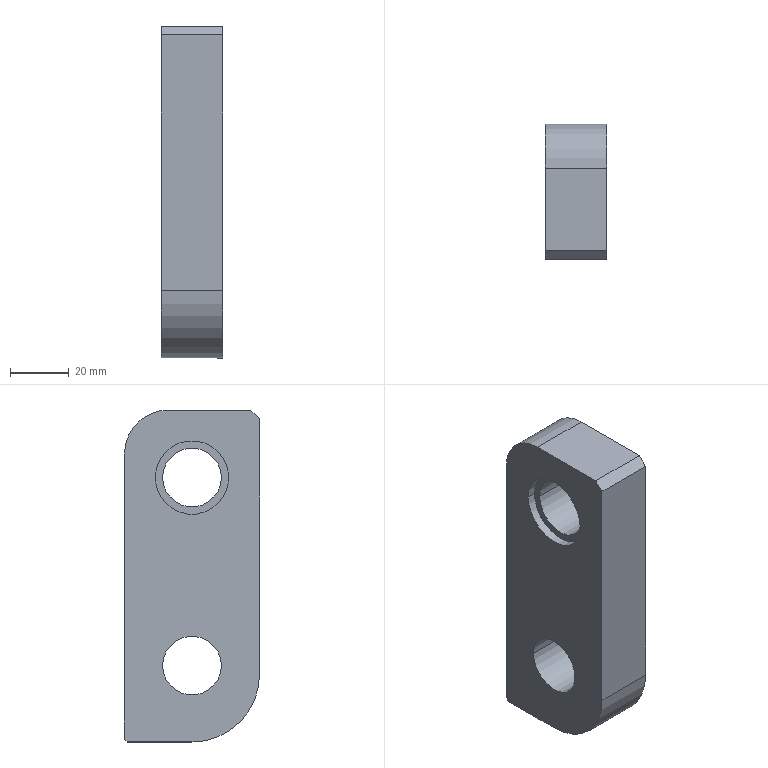Component | SolidWorks | GL9-255--p_O(_k)-1 | 1 solid | 17 faces | box 21 x 46 x 113 mm | volume 91930 mm3 | plane 9 | cylinder 8 | commonest cylinder face diameters 20 x4 25 x2 30 x1 46 x1
build123d program:
from build123d import *

# Parameters (mm, degrees)
SKETCH1_W      = 113
SKETCH1_H      = 46
EXTRUDE1_DEPTH = 21
FILLET1_R      = 15
FILLET2_R      = 23
SKETCH2_R      = 10
EXTRUDE2_DEPTH = 124.798
CHAMFER1_SIZE  = 3
CHAMFER2_SIZE  = 1
SKETCH4_R      = 12.5
EXTRUDE4_DEPTH = 3
SKETCH5_R      = 10
EXTRUDE5_DEPTH = 124.325


with BuildPart() as part:
    # Sketch1 → Extrude1 (new body)
    with BuildSketch(Plane(origin=(0, 0, 0), x_dir=(1, 0, 0), z_dir=(0, 1, 0))):
        with Locations((-56.5, -23)):
            Rectangle(SKETCH1_W, SKETCH1_H)
    extrude(amount=EXTRUDE1_DEPTH)

    # Fillet1
    fillet1_edges = [part.edges().sort_by_distance(p)[0] for p in [
        (-113, 10.5, 0),
    ]]
    fillet(fillet1_edges, radius=FILLET1_R)

    # Fillet2
    fillet2_edges = [part.edges().sort_by_distance(p)[0] for p in [
        (0, 10.5, 46),
    ]]
    fillet(fillet2_edges, radius=FILLET2_R)

    # Sketch2 → Extrude2 (cut, through all)
    with BuildSketch(Plane(origin=(0, 21, 0), x_dir=(1, 0, 0), z_dir=(0, 1, 0))):
        with Locations(Location((-26, -23, 0), (0, 0, 270))):
            Circle(SKETCH2_R)
    extrude(amount=-EXTRUDE2_DEPTH, mode=Mode.SUBTRACT)

    # Chamfer1
    chamfer1_edges = [part.edges().sort_by_distance(p)[0] for p in [
        (-113, 10.5, 46),
    ]]
    chamfer(chamfer1_edges, length=CHAMFER1_SIZE)

    # Chamfer2
    chamfer2_edges = [part.edges().sort_by_distance(p)[0] for p in [
        (0, 10.5, 0),
    ]]
    chamfer(chamfer2_edges, length=CHAMFER2_SIZE)

    # Sketch4 → Extrude4 (cut)
    with BuildSketch(Plane.XZ):
        with Locations(Location((-90, 23, 0), (0, 0, 270))):
            Circle(SKETCH4_R)
    extrude(amount=-EXTRUDE4_DEPTH, mode=Mode.SUBTRACT)

    # Sketch5 → Extrude5 (cut, through all)
    with BuildSketch(Plane.XZ.offset(-3)):
        with Locations(Location((-90, 23, 0), (0, 0, 270))):
            Circle(SKETCH5_R)
    extrude(amount=-EXTRUDE5_DEPTH, mode=Mode.SUBTRACT)


solid = part.part

# Placed as in the assembly
solid = solid.moved(Location((64, 104, -550), (90, 0, -90)))
STEP:
#1=COLOUR_RGB('',0.7922,0.8196,0.9333);
#2=FILL_AREA_STYLE_COLOUR('',#1);
#3=FILL_AREA_STYLE('',(#2));
#4=SURFACE_STYLE_FILL_AREA(#3);
#5=SURFACE_SIDE_STYLE('',(#4));
#6=SURFACE_STYLE_USAGE(.BOTH.,#5);
#7=PRESENTATION_STYLE_ASSIGNMENT((#6));
#8=CARTESIAN_POINT('',(3.346,2.795,-18.11));
#9=VERTEX_POINT('',#8);
#10=CARTESIAN_POINT('',(3.346,3.583,-18.11));
#11=VERTEX_POINT('',#10);
#12=CARTESIAN_POINT('',(3.346,3.189,-18.11));
#13=DIRECTION('',(-1.,0.,0.));
#14=DIRECTION('',(0.,1.,0.));
#15=AXIS2_PLACEMENT_3D('',#12,#13,#14);
#16=CIRCLE('',#15,0.3937);
#17=EDGE_CURVE('',#9,#11,#16,.T.);
#18=ORIENTED_EDGE('',*,*,#17,.F.);
#19=CARTESIAN_POINT('',(2.638,2.795,-18.11));
#20=VERTEX_POINT('',#19);
#21=CARTESIAN_POINT('',(3.346,2.795,-18.11));
#22=DIRECTION('',(-1.,0.,0.));
#23=VECTOR('',#22,39.37);
#24=LINE('',#21,#23);
#25=EDGE_CURVE('',#9,#20,#24,.T.);
#26=ORIENTED_EDGE('',*,*,#25,.T.);
#27=CARTESIAN_POINT('',(2.638,3.583,-18.11));
#28=VERTEX_POINT('',#27);
#29=CARTESIAN_POINT('',(2.638,3.189,-18.11));
#30=DIRECTION('',(-1.,0.,0.));
#31=DIRECTION('',(0.,1.,0.));
#32=AXIS2_PLACEMENT_3D('',#29,#30,#31);
#33=CIRCLE('',#32,0.3937);
#34=EDGE_CURVE('',#20,#28,#33,.T.);
#35=ORIENTED_EDGE('',*,*,#34,.T.);
#36=CARTESIAN_POINT('',(3.346,3.583,-18.11));
#37=DIRECTION('',(-1.,0.,0.));
#38=VECTOR('',#37,39.37);
#39=LINE('',#36,#38);
#40=EDGE_CURVE('',#11,#28,#39,.T.);
#41=ORIENTED_EDGE('',*,*,#40,.F.);
#42=EDGE_LOOP('',(#18,#26,#35,#41));
#43=FACE_OUTER_BOUND('',#42,.T.);
#44=CARTESIAN_POINT('',(3.346,3.189,-18.11));
#45=DIRECTION('',(-1.,0.,0.));
#46=DIRECTION('',(0.,1.,0.));
#47=AXIS2_PLACEMENT_3D('',#44,#45,#46);
#48=CYLINDRICAL_SURFACE('',#47,0.3937);
#49=ADVANCED_FACE('',(#43),#48,.F.);
#50=CARTESIAN_POINT('',(2.638,2.697,-18.11));
#51=VERTEX_POINT('',#50);
#52=CARTESIAN_POINT('',(2.638,3.681,-18.11));
#53=VERTEX_POINT('',#52);
#54=CARTESIAN_POINT('',(2.638,3.189,-18.11));
#55=DIRECTION('',(-1.,0.,0.));
#56=DIRECTION('',(0.,1.,0.));
#57=AXIS2_PLACEMENT_3D('',#54,#55,#56);
#58=CIRCLE('',#57,0.4921);
#59=EDGE_CURVE('',#51,#53,#58,.T.);
#60=ORIENTED_EDGE('',*,*,#59,.F.);
#61=CARTESIAN_POINT('',(2.52,2.697,-18.11));
#62=VERTEX_POINT('',#61);
#63=CARTESIAN_POINT('',(2.638,2.697,-18.11));
#64=DIRECTION('',(-1.,0.,0.));
#65=VECTOR('',#64,39.37);
#66=LINE('',#63,#65);
#67=EDGE_CURVE('',#51,#62,#66,.T.);
#68=ORIENTED_EDGE('',*,*,#67,.T.);
#69=CARTESIAN_POINT('',(2.52,3.681,-18.11));
#70=VERTEX_POINT('',#69);
#71=CARTESIAN_POINT('',(2.52,3.189,-18.11));
#72=DIRECTION('',(-1.,0.,0.));
#73=DIRECTION('',(0.,1.,0.));
#74=AXIS2_PLACEMENT_3D('',#71,#72,#73);
#75=CIRCLE('',#74,0.4921);
#76=EDGE_CURVE('',#62,#70,#75,.T.);
#77=ORIENTED_EDGE('',*,*,#76,.T.);
#78=CARTESIAN_POINT('',(2.638,3.681,-18.11));
#79=DIRECTION('',(-1.,0.,0.));
#80=VECTOR('',#79,39.37);
#81=LINE('',#78,#80);
#82=EDGE_CURVE('',#53,#70,#81,.T.);
#83=ORIENTED_EDGE('',*,*,#82,.F.);
#84=EDGE_LOOP('',(#60,#68,#77,#83));
#85=FACE_OUTER_BOUND('',#84,.T.);
#86=CARTESIAN_POINT('',(2.638,3.189,-18.11));
#87=DIRECTION('',(-1.,0.,0.));
#88=DIRECTION('',(0.,1.,0.));
#89=AXIS2_PLACEMENT_3D('',#86,#87,#88);
#90=CYLINDRICAL_SURFACE('',#89,0.4921);
#91=ADVANCED_FACE('',(#85),#90,.F.);
#92=CARTESIAN_POINT('',(2.52,3.583,-20.63));
#93=VERTEX_POINT('',#92);
#94=CARTESIAN_POINT('',(2.52,2.795,-20.63));
#95=VERTEX_POINT('',#94);
#96=CARTESIAN_POINT('',(2.52,3.189,-20.63));
#97=DIRECTION('',(1.,-0.,-0.));
#98=DIRECTION('',(0.,-1.,0.));
#99=AXIS2_PLACEMENT_3D('',#96,#97,#98);
#100=CIRCLE('',#99,0.3937);
#101=EDGE_CURVE('',#93,#95,#100,.T.);
#102=ORIENTED_EDGE('',*,*,#101,.F.);
#103=CARTESIAN_POINT('',(3.346,3.583,-20.63));
#104=VERTEX_POINT('',#103);
#105=CARTESIAN_POINT('',(2.52,3.583,-20.63));
#106=DIRECTION('',(1.,-0.,-0.));
#107=VECTOR('',#106,39.37);
#108=LINE('',#105,#107);
#109=EDGE_CURVE('',#93,#104,#108,.T.);
#110=ORIENTED_EDGE('',*,*,#109,.T.);
#111=CARTESIAN_POINT('',(3.346,2.795,-20.63));
#112=VERTEX_POINT('',#111);
#113=CARTESIAN_POINT('',(3.346,3.189,-20.63));
#114=DIRECTION('',(1.,-0.,-0.));
#115=DIRECTION('',(0.,-1.,0.));
#116=AXIS2_PLACEMENT_3D('',#113,#114,#115);
#117=CIRCLE('',#116,0.3937);
#118=EDGE_CURVE('',#104,#112,#117,.T.);
#119=ORIENTED_EDGE('',*,*,#118,.T.);
#120=CARTESIAN_POINT('',(2.52,2.795,-20.63));
#121=DIRECTION('',(1.,-0.,-0.));
#122=VECTOR('',#121,39.37);
#123=LINE('',#120,#122);
#124=EDGE_CURVE('',#95,#112,#123,.T.);
#125=ORIENTED_EDGE('',*,*,#124,.F.);
#126=EDGE_LOOP('',(#102,#110,#119,#125));
#127=FACE_OUTER_BOUND('',#126,.T.);
#128=CARTESIAN_POINT('',(2.52,3.189,-20.63));
#129=DIRECTION('',(1.,-0.,-0.));
#130=DIRECTION('',(0.,-1.,0.));
#131=AXIS2_PLACEMENT_3D('',#128,#129,#130);
#132=CYLINDRICAL_SURFACE('',#131,0.3937);
#133=ADVANCED_FACE('',(#127),#132,.F.);
#134=CARTESIAN_POINT('',(2.52,3.189,-21.654));
#135=VERTEX_POINT('',#134);
#136=CARTESIAN_POINT('',(2.52,4.055,-21.654));
#137=VERTEX_POINT('',#136);
#138=CARTESIAN_POINT('',(2.52,2.283,-21.654));
#139=DIRECTION('',(0.,1.,0.));
#140=VECTOR('',#139,39.37);
#141=LINE('',#138,#140);
#142=EDGE_CURVE('',#135,#137,#141,.T.);
#143=ORIENTED_EDGE('',*,*,#142,.T.);
#144=CARTESIAN_POINT('',(3.346,4.055,-21.654));
#145=VERTEX_POINT('',#144);
#146=CARTESIAN_POINT('',(3.346,4.055,-21.654));
#147=DIRECTION('',(1.,-0.,-0.));
#148=VECTOR('',#147,39.37);
#149=LINE('',#146,#148);
#150=EDGE_CURVE('',#137,#145,#149,.T.);
#151=ORIENTED_EDGE('',*,*,#150,.T.);
#152=CARTESIAN_POINT('',(3.346,3.189,-21.654));
#153=VERTEX_POINT('',#152);
#154=CARTESIAN_POINT('',(3.346,2.283,-21.654));
#155=DIRECTION('',(0.,1.,0.));
#156=VECTOR('',#155,39.37);
#157=LINE('',#154,#156);
#158=EDGE_CURVE('',#153,#145,#157,.T.);
#159=ORIENTED_EDGE('',*,*,#158,.F.);
#160=CARTESIAN_POINT('',(3.346,3.189,-21.654));
#161=DIRECTION('',(-1.,0.,0.));
#162=VECTOR('',#161,39.37);
#163=LINE('',#160,#162);
#164=EDGE_CURVE('',#153,#135,#163,.T.);
#165=ORIENTED_EDGE('',*,*,#164,.T.);
#166=EDGE_LOOP('',(#143,#151,#159,#165));
#167=FACE_OUTER_BOUND('',#166,.T.);
#168=CARTESIAN_POINT('',(3.346,2.283,-21.654));
#169=DIRECTION('',(0.,-0.,1.));
#170=DIRECTION('',(-0.,-1.,-0.));
#171=AXIS2_PLACEMENT_3D('',#168,#169,#170);
#172=PLANE('',#171);
#173=ADVANCED_FACE('',(#167),#172,.F.);
#174=CARTESIAN_POINT('',(3.346,4.094,-21.614));
#175=VERTEX_POINT('',#174);
#176=CARTESIAN_POINT('',(3.346,4.094,-17.795));
#177=VERTEX_POINT('',#176);
#178=CARTESIAN_POINT('',(3.346,4.094,-21.654));
#179=DIRECTION('',(0.,-0.,1.));
#180=VECTOR('',#179,39.37);
#181=LINE('',#178,#180);
#182=EDGE_CURVE('',#175,#177,#181,.T.);
#183=ORIENTED_EDGE('',*,*,#182,.F.);
#184=CARTESIAN_POINT('',(2.52,4.094,-21.614));
#185=VERTEX_POINT('',#184);
#186=CARTESIAN_POINT('',(3.346,4.094,-21.614));
#187=DIRECTION('',(-1.,0.,0.));
#188=VECTOR('',#187,39.37);
#189=LINE('',#186,#188);
#190=EDGE_CURVE('',#175,#185,#189,.T.);
#191=ORIENTED_EDGE('',*,*,#190,.T.);
#192=CARTESIAN_POINT('',(2.52,4.094,-17.795));
#193=VERTEX_POINT('',#192);
#194=CARTESIAN_POINT('',(2.52,4.094,-21.654));
#195=DIRECTION('',(0.,-0.,1.));
#196=VECTOR('',#195,39.37);
#197=LINE('',#194,#196);
#198=EDGE_CURVE('',#185,#193,#197,.T.);
#199=ORIENTED_EDGE('',*,*,#198,.T.);
#200=CARTESIAN_POINT('',(3.346,4.094,-17.795));
#201=DIRECTION('',(1.,-0.,-0.));
#202=VECTOR('',#201,39.37);
#203=LINE('',#200,#202);
#204=EDGE_CURVE('',#193,#177,#203,.T.);
#205=ORIENTED_EDGE('',*,*,#204,.T.);
#206=EDGE_LOOP('',(#183,#191,#199,#205));
#207=FACE_OUTER_BOUND('',#206,.T.);
#208=CARTESIAN_POINT('',(3.346,4.094,-21.654));
#209=DIRECTION('',(-0.,-1.,-0.));
#210=DIRECTION('',(-0.,0.,-1.));
#211=AXIS2_PLACEMENT_3D('',#208,#209,#210);
#212=PLANE('',#211);
#213=ADVANCED_FACE('',(#207),#212,.F.);
#214=CARTESIAN_POINT('',(2.52,3.504,-17.205));
#215=VERTEX_POINT('',#214);
#216=CARTESIAN_POINT('',(2.52,2.402,-17.205));
#217=VERTEX_POINT('',#216);
#218=CARTESIAN_POINT('',(2.52,4.094,-17.205));
#219=DIRECTION('',(-0.,-1.,-0.));
#220=VECTOR('',#219,39.37);
#221=LINE('',#218,#220);
#222=EDGE_CURVE('',#215,#217,#221,.T.);
#223=ORIENTED_EDGE('',*,*,#222,.T.);
#224=CARTESIAN_POINT('',(3.346,2.402,-17.205));
#225=VERTEX_POINT('',#224);
#226=CARTESIAN_POINT('',(3.346,2.402,-17.205));
#227=DIRECTION('',(1.,-0.,-0.));
#228=VECTOR('',#227,39.37);
#229=LINE('',#226,#228);
#230=EDGE_CURVE('',#217,#225,#229,.T.);
#231=ORIENTED_EDGE('',*,*,#230,.T.);
#232=CARTESIAN_POINT('',(3.346,3.504,-17.205));
#233=VERTEX_POINT('',#232);
#234=CARTESIAN_POINT('',(3.346,4.094,-17.205));
#235=DIRECTION('',(-0.,-1.,-0.));
#236=VECTOR('',#235,39.37);
#237=LINE('',#234,#236);
#238=EDGE_CURVE('',#233,#225,#237,.T.);
#239=ORIENTED_EDGE('',*,*,#238,.F.);
#240=CARTESIAN_POINT('',(3.346,3.504,-17.205));
#241=DIRECTION('',(-1.,0.,0.));
#242=VECTOR('',#241,39.37);
#243=LINE('',#240,#242);
#244=EDGE_CURVE('',#233,#215,#243,.T.);
#245=ORIENTED_EDGE('',*,*,#244,.T.);
#246=EDGE_LOOP('',(#223,#231,#239,#245));
#247=FACE_OUTER_BOUND('',#246,.T.);
#248=CARTESIAN_POINT('',(3.346,4.094,-17.205));
#249=DIRECTION('',(-0.,0.,-1.));
#250=DIRECTION('',(0.,1.,0.));
#251=AXIS2_PLACEMENT_3D('',#248,#249,#250);
#252=PLANE('',#251);
#253=ADVANCED_FACE('',(#247),#252,.F.);
#254=CARTESIAN_POINT('',(3.346,2.283,-17.323));
#255=VERTEX_POINT('',#254);
#256=CARTESIAN_POINT('',(3.346,2.283,-20.748));
#257=VERTEX_POINT('',#256);
#258=CARTESIAN_POINT('',(3.346,2.283,-17.205));
#259=DIRECTION('',(-0.,0.,-1.));
#260=VECTOR('',#259,39.37);
#261=LINE('',#258,#260);
#262=EDGE_CURVE('',#255,#257,#261,.T.);
#263=ORIENTED_EDGE('',*,*,#262,.F.);
#264=CARTESIAN_POINT('',(2.52,2.283,-17.323));
#265=VERTEX_POINT('',#264);
#266=CARTESIAN_POINT('',(3.346,2.283,-17.323));
#267=DIRECTION('',(-1.,0.,0.));
#268=VECTOR('',#267,39.37);
#269=LINE('',#266,#268);
#270=EDGE_CURVE('',#255,#265,#269,.T.);
#271=ORIENTED_EDGE('',*,*,#270,.T.);
#272=CARTESIAN_POINT('',(2.52,2.283,-20.748));
#273=VERTEX_POINT('',#272);
#274=CARTESIAN_POINT('',(2.52,2.283,-17.205));
#275=DIRECTION('',(-0.,0.,-1.));
#276=VECTOR('',#275,39.37);
#277=LINE('',#274,#276);
#278=EDGE_CURVE('',#265,#273,#277,.T.);
#279=ORIENTED_EDGE('',*,*,#278,.T.);
#280=CARTESIAN_POINT('',(3.346,2.283,-20.748));
#281=DIRECTION('',(1.,-0.,-0.));
#282=VECTOR('',#281,39.37);
#283=LINE('',#280,#282);
#284=EDGE_CURVE('',#273,#257,#283,.T.);
#285=ORIENTED_EDGE('',*,*,#284,.T.);
#286=EDGE_LOOP('',(#263,#271,#279,#285));
#287=FACE_OUTER_BOUND('',#286,.T.);
#288=CARTESIAN_POINT('',(3.346,2.283,-17.205));
#289=DIRECTION('',(0.,1.,0.));
#290=DIRECTION('',(0.,-0.,1.));
#291=AXIS2_PLACEMENT_3D('',#288,#289,#290);
#292=PLANE('',#291);
#293=ADVANCED_FACE('',(#287),#292,.F.);
#294=CARTESIAN_POINT('',(3.346,3.189,-18.11));
#295=DIRECTION('',(-1.,0.,0.));
#296=DIRECTION('',(0.,1.,0.));
#297=AXIS2_PLACEMENT_3D('',#294,#295,#296);
#298=CIRCLE('',#297,0.3937);
#299=EDGE_CURVE('',#11,#9,#298,.T.);
#300=ORIENTED_EDGE('',*,*,#299,.T.);
#301=ORIENTED_EDGE('',*,*,#17,.T.);
#302=EDGE_LOOP('',(#300,#301));
#303=FACE_BOUND('',#302,.T.);
#304=CARTESIAN_POINT('',(3.346,3.189,-20.63));
#305=DIRECTION('',(1.,-0.,-0.));
#306=DIRECTION('',(0.,-1.,0.));
#307=AXIS2_PLACEMENT_3D('',#304,#305,#306);
#308=CIRCLE('',#307,0.3937);
#309=EDGE_CURVE('',#112,#104,#308,.T.);
#310=ORIENTED_EDGE('',*,*,#309,.F.);
#311=ORIENTED_EDGE('',*,*,#118,.F.);
#312=EDGE_LOOP('',(#310,#311));
#313=FACE_BOUND('',#312,.T.);
#314=ORIENTED_EDGE('',*,*,#158,.T.);
#315=CARTESIAN_POINT('',(3.346,4.075,-21.634));
#316=DIRECTION('',(0.,0.7071,0.7071));
#317=VECTOR('',#316,39.37);
#318=LINE('',#315,#317);
#319=EDGE_CURVE('',#145,#175,#318,.T.);
#320=ORIENTED_EDGE('',*,*,#319,.T.);
#321=ORIENTED_EDGE('',*,*,#182,.T.);
#322=CARTESIAN_POINT('',(3.346,3.504,-17.795));
#323=DIRECTION('',(1.,-0.,-0.));
#324=DIRECTION('',(0.,-1.,0.));
#325=AXIS2_PLACEMENT_3D('',#322,#323,#324);
#326=CIRCLE('',#325,0.5906);
#327=EDGE_CURVE('',#177,#233,#326,.T.);
#328=ORIENTED_EDGE('',*,*,#327,.T.);
#329=ORIENTED_EDGE('',*,*,#238,.T.);
#330=CARTESIAN_POINT('',(3.346,1.024,-18.583));
#331=DIRECTION('',(-0.,-0.7071,-0.7071));
#332=VECTOR('',#331,39.37);
#333=LINE('',#330,#332);
#334=EDGE_CURVE('',#225,#255,#333,.T.);
#335=ORIENTED_EDGE('',*,*,#334,.T.);
#336=ORIENTED_EDGE('',*,*,#262,.T.);
#337=CARTESIAN_POINT('',(3.346,3.189,-20.748));
#338=DIRECTION('',(1.,-0.,-0.));
#339=DIRECTION('',(0.,-1.,0.));
#340=AXIS2_PLACEMENT_3D('',#337,#338,#339);
#341=CIRCLE('',#340,0.9055);
#342=EDGE_CURVE('',#257,#153,#341,.T.);
#343=ORIENTED_EDGE('',*,*,#342,.T.);
#344=EDGE_LOOP('',(#314,#320,#321,#328,#329,#335,#336,#343));
#345=FACE_OUTER_BOUND('',#344,.T.);
#346=CARTESIAN_POINT('',(3.346,4.094,-21.654));
#347=DIRECTION('',(1.,0.,-0.));
#348=DIRECTION('',(-0.,-1.,-0.));
#349=AXIS2_PLACEMENT_3D('',#346,#347,#348);
#350=PLANE('',#349);
#351=ADVANCED_FACE('',(#303,#313,#345),#350,.T.);
#352=CARTESIAN_POINT('',(2.52,3.189,-18.11));
#353=DIRECTION('',(-1.,0.,0.));
#354=DIRECTION('',(0.,1.,0.));
#355=AXIS2_PLACEMENT_3D('',#352,#353,#354);
#356=CIRCLE('',#355,0.4921);
#357=EDGE_CURVE('',#70,#62,#356,.T.);
#358=ORIENTED_EDGE('',*,*,#357,.F.);
#359=ORIENTED_EDGE('',*,*,#76,.F.);
#360=EDGE_LOOP('',(#358,#359));
#361=FACE_BOUND('',#360,.T.);
#362=CARTESIAN_POINT('',(2.52,3.189,-20.63));
#363=DIRECTION('',(1.,-0.,-0.));
#364=DIRECTION('',(0.,-1.,0.));
#365=AXIS2_PLACEMENT_3D('',#362,#363,#364);
#366=CIRCLE('',#365,0.3937);
#367=EDGE_CURVE('',#95,#93,#366,.T.);
#368=ORIENTED_EDGE('',*,*,#367,.T.);
#369=ORIENTED_EDGE('',*,*,#101,.T.);
#370=EDGE_LOOP('',(#368,#369));
#371=FACE_BOUND('',#370,.T.);
#372=ORIENTED_EDGE('',*,*,#198,.F.);
#373=CARTESIAN_POINT('',(2.52,4.094,-21.614));
#374=DIRECTION('',(-0.,-0.7071,-0.7071));
#375=VECTOR('',#374,39.37);
#376=LINE('',#373,#375);
#377=EDGE_CURVE('',#185,#137,#376,.T.);
#378=ORIENTED_EDGE('',*,*,#377,.T.);
#379=ORIENTED_EDGE('',*,*,#142,.F.);
#380=CARTESIAN_POINT('',(2.52,3.189,-20.748));
#381=DIRECTION('',(-1.,0.,0.));
#382=DIRECTION('',(0.,-1.,0.));
#383=AXIS2_PLACEMENT_3D('',#380,#381,#382);
#384=CIRCLE('',#383,0.9055);
#385=EDGE_CURVE('',#135,#273,#384,.T.);
#386=ORIENTED_EDGE('',*,*,#385,.T.);
#387=ORIENTED_EDGE('',*,*,#278,.F.);
#388=CARTESIAN_POINT('',(2.52,2.283,-17.323));
#389=DIRECTION('',(0.,0.7071,0.7071));
#390=VECTOR('',#389,39.37);
#391=LINE('',#388,#390);
#392=EDGE_CURVE('',#265,#217,#391,.T.);
#393=ORIENTED_EDGE('',*,*,#392,.T.);
#394=ORIENTED_EDGE('',*,*,#222,.F.);
#395=CARTESIAN_POINT('',(2.52,3.504,-17.795));
#396=DIRECTION('',(-1.,0.,0.));
#397=DIRECTION('',(0.,-1.,-0.));
#398=AXIS2_PLACEMENT_3D('',#395,#396,#397);
#399=CIRCLE('',#398,0.5906);
#400=EDGE_CURVE('',#215,#193,#399,.T.);
#401=ORIENTED_EDGE('',*,*,#400,.T.);
#402=EDGE_LOOP('',(#372,#378,#379,#386,#387,#393,#394,#401));
#403=FACE_OUTER_BOUND('',#402,.T.);
#404=CARTESIAN_POINT('',(2.52,4.094,-21.654));
#405=DIRECTION('',(1.,0.,-0.));
#406=DIRECTION('',(-0.,-1.,-0.));
#407=AXIS2_PLACEMENT_3D('',#404,#405,#406);
#408=PLANE('',#407);
#409=ADVANCED_FACE('',(#361,#371,#403),#408,.F.);
#410=ORIENTED_EDGE('',*,*,#327,.F.);
#411=ORIENTED_EDGE('',*,*,#204,.F.);
#412=ORIENTED_EDGE('',*,*,#400,.F.);
#413=ORIENTED_EDGE('',*,*,#244,.F.);
#414=EDGE_LOOP('',(#410,#411,#412,#413));
#415=FACE_OUTER_BOUND('',#414,.T.);
#416=CARTESIAN_POINT('',(3.346,3.504,-17.795));
#417=DIRECTION('',(-1.,0.,0.));
#418=DIRECTION('',(0.,1.,0.));
#419=AXIS2_PLACEMENT_3D('',#416,#417,#418);
#420=CYLINDRICAL_SURFACE('',#419,0.5906);
#421=ADVANCED_FACE('',(#415),#420,.T.);
#422=ORIENTED_EDGE('',*,*,#342,.F.);
#423=ORIENTED_EDGE('',*,*,#284,.F.);
#424=ORIENTED_EDGE('',*,*,#385,.F.);
#425=ORIENTED_EDGE('',*,*,#164,.F.);
#426=EDGE_LOOP('',(#422,#423,#424,#425));
#427=FACE_OUTER_BOUND('',#426,.T.);
#428=CARTESIAN_POINT('',(3.346,3.189,-20.748));
#429=DIRECTION('',(-1.,0.,0.));
#430=DIRECTION('',(0.,1.,0.));
#431=AXIS2_PLACEMENT_3D('',#428,#429,#430);
#432=CYLINDRICAL_SURFACE('',#431,0.9055);
#433=ADVANCED_FACE('',(#427),#432,.T.);
#434=ORIENTED_EDGE('',*,*,#109,.F.);
#435=ORIENTED_EDGE('',*,*,#367,.F.);
#436=ORIENTED_EDGE('',*,*,#124,.T.);
#437=ORIENTED_EDGE('',*,*,#309,.T.);
#438=EDGE_LOOP('',(#434,#435,#436,#437));
#439=FACE_OUTER_BOUND('',#438,.T.);
#440=CARTESIAN_POINT('',(2.52,3.189,-20.63));
#441=DIRECTION('',(1.,-0.,-0.));
#442=DIRECTION('',(0.,-1.,0.));
#443=AXIS2_PLACEMENT_3D('',#440,#441,#442);
#444=CYLINDRICAL_SURFACE('',#443,0.3937);
#445=ADVANCED_FACE('',(#439),#444,.F.);
#446=ORIENTED_EDGE('',*,*,#334,.F.);
#447=ORIENTED_EDGE('',*,*,#230,.F.);
#448=ORIENTED_EDGE('',*,*,#392,.F.);
#449=ORIENTED_EDGE('',*,*,#270,.F.);
#450=EDGE_LOOP('',(#446,#447,#448,#449));
#451=FACE_OUTER_BOUND('',#450,.T.);
#452=CARTESIAN_POINT('',(3.346,2.283,-17.323));
#453=DIRECTION('',(-0.,0.7071,-0.7071));
#454=DIRECTION('',(0.,0.7071,0.7071));
#455=AXIS2_PLACEMENT_3D('',#452,#453,#454);
#456=PLANE('',#455);
#457=ADVANCED_FACE('',(#451),#456,.F.);
#458=ORIENTED_EDGE('',*,*,#319,.F.);
#459=ORIENTED_EDGE('',*,*,#150,.F.);
#460=ORIENTED_EDGE('',*,*,#377,.F.);
#461=ORIENTED_EDGE('',*,*,#190,.F.);
#462=EDGE_LOOP('',(#458,#459,#460,#461));
#463=FACE_OUTER_BOUND('',#462,.T.);
#464=CARTESIAN_POINT('',(3.346,4.094,-21.614));
#465=DIRECTION('',(0.,-0.7071,0.7071));
#466=DIRECTION('',(-0.,-0.7071,-0.7071));
#467=AXIS2_PLACEMENT_3D('',#464,#465,#466);
#468=PLANE('',#467);
#469=ADVANCED_FACE('',(#463),#468,.F.);
#470=ORIENTED_EDGE('',*,*,#67,.F.);
#471=CARTESIAN_POINT('',(2.638,3.189,-18.11));
#472=DIRECTION('',(-1.,0.,0.));
#473=DIRECTION('',(0.,1.,0.));
#474=AXIS2_PLACEMENT_3D('',#471,#472,#473);
#475=CIRCLE('',#474,0.4921);
#476=EDGE_CURVE('',#53,#51,#475,.T.);
#477=ORIENTED_EDGE('',*,*,#476,.F.);
#478=ORIENTED_EDGE('',*,*,#82,.T.);
#479=ORIENTED_EDGE('',*,*,#357,.T.);
#480=EDGE_LOOP('',(#470,#477,#478,#479));
#481=FACE_OUTER_BOUND('',#480,.T.);
#482=CARTESIAN_POINT('',(2.638,3.189,-18.11));
#483=DIRECTION('',(-1.,0.,0.));
#484=DIRECTION('',(0.,1.,0.));
#485=AXIS2_PLACEMENT_3D('',#482,#483,#484);
#486=CYLINDRICAL_SURFACE('',#485,0.4921);
#487=ADVANCED_FACE('',(#481),#486,.F.);
#488=CARTESIAN_POINT('',(2.638,3.189,-18.11));
#489=DIRECTION('',(-1.,0.,0.));
#490=DIRECTION('',(0.,1.,0.));
#491=AXIS2_PLACEMENT_3D('',#488,#489,#490);
#492=CIRCLE('',#491,0.3937);
#493=EDGE_CURVE('',#28,#20,#492,.T.);
#494=ORIENTED_EDGE('',*,*,#493,.F.);
#495=ORIENTED_EDGE('',*,*,#34,.F.);
#496=EDGE_LOOP('',(#494,#495));
#497=FACE_BOUND('',#496,.T.);
#498=ORIENTED_EDGE('',*,*,#476,.T.);
#499=ORIENTED_EDGE('',*,*,#59,.T.);
#500=EDGE_LOOP('',(#498,#499));
#501=FACE_OUTER_BOUND('',#500,.T.);
#502=CARTESIAN_POINT('',(2.638,3.189,-18.11));
#503=DIRECTION('',(-1.,-0.,0.));
#504=DIRECTION('',(0.,1.,0.));
#505=AXIS2_PLACEMENT_3D('',#502,#503,#504);
#506=PLANE('',#505);
#507=ADVANCED_FACE('',(#497,#501),#506,.T.);
#508=ORIENTED_EDGE('',*,*,#25,.F.);
#509=ORIENTED_EDGE('',*,*,#299,.F.);
#510=ORIENTED_EDGE('',*,*,#40,.T.);
#511=ORIENTED_EDGE('',*,*,#493,.T.);
#512=EDGE_LOOP('',(#508,#509,#510,#511));
#513=FACE_OUTER_BOUND('',#512,.T.);
#514=CARTESIAN_POINT('',(3.346,3.189,-18.11));
#515=DIRECTION('',(-1.,0.,0.));
#516=DIRECTION('',(0.,1.,0.));
#517=AXIS2_PLACEMENT_3D('',#514,#515,#516);
#518=CYLINDRICAL_SURFACE('',#517,0.3937);
#519=ADVANCED_FACE('',(#513),#518,.F.);
#520=CLOSED_SHELL('',(#49,#91,#133,#173,#213,#253,#293,#351,#409,#421,#433,#445,#457,#469,#487,#507,#519));
#521=MANIFOLD_SOLID_BREP('',#520);
#522=STYLED_ITEM('',(#7),#521);
#523=PRESENTATION_LAYER_ASSIGNMENT('','',(#522));
#524=CARTESIAN_POINT('',(0.,0.,0.));
#525=DIRECTION('',(0.,0.,1.));
#526=DIRECTION('',(1.,0.,0.));
#527=AXIS2_PLACEMENT_3D('',#524,#525,#526);
#528=(LENGTH_UNIT()NAMED_UNIT(*)SI_UNIT($,.METRE.));
#529=LENGTH_MEASURE_WITH_UNIT(LENGTH_MEASURE(0.0254),#528);
#530=DIMENSIONAL_EXPONENTS(1.,0.,0.,0.,0.,0.,0.);
#531=(CONVERSION_BASED_UNIT('',#529)LENGTH_UNIT()NAMED_UNIT(#530));
#532=UNCERTAINTY_MEASURE_WITH_UNIT(LENGTH_MEASURE(0.00001),#531,'','');
#533=(NAMED_UNIT(*)PLANE_ANGLE_UNIT()SI_UNIT($,.RADIAN.));
#534=(NAMED_UNIT(*)SI_UNIT($,.STERADIAN.)SOLID_ANGLE_UNIT());
#535=(GEOMETRIC_REPRESENTATION_CONTEXT(3)GLOBAL_UNCERTAINTY_ASSIGNED_CONTEXT((#532))GLOBAL_UNIT_ASSIGNED_CONTEXT((#531,#533,#534))REPRESENTATION_CONTEXT('',''));
#536=ADVANCED_BREP_SHAPE_REPRESENTATION('',(#521,#527),#535);
#537=(LENGTH_UNIT()NAMED_UNIT(*)SI_UNIT($,.METRE.));
#538=LENGTH_MEASURE_WITH_UNIT(LENGTH_MEASURE(0.0254),#537);
#539=DIMENSIONAL_EXPONENTS(1.,0.,0.,0.,0.,0.,0.);
#540=(CONVERSION_BASED_UNIT('',#538)LENGTH_UNIT()NAMED_UNIT(#539));
#541=UNCERTAINTY_MEASURE_WITH_UNIT(LENGTH_MEASURE(0.00001),#540,'','');
#542=(NAMED_UNIT(*)PLANE_ANGLE_UNIT()SI_UNIT($,.RADIAN.));
#543=(NAMED_UNIT(*)SI_UNIT($,.STERADIAN.)SOLID_ANGLE_UNIT());
#544=(GEOMETRIC_REPRESENTATION_CONTEXT(3)GLOBAL_UNCERTAINTY_ASSIGNED_CONTEXT((#541))GLOBAL_UNIT_ASSIGNED_CONTEXT((#540,#542,#543))REPRESENTATION_CONTEXT('',''));
#545=MECHANICAL_DESIGN_GEOMETRIC_PRESENTATION_REPRESENTATION('',(#522),#544);